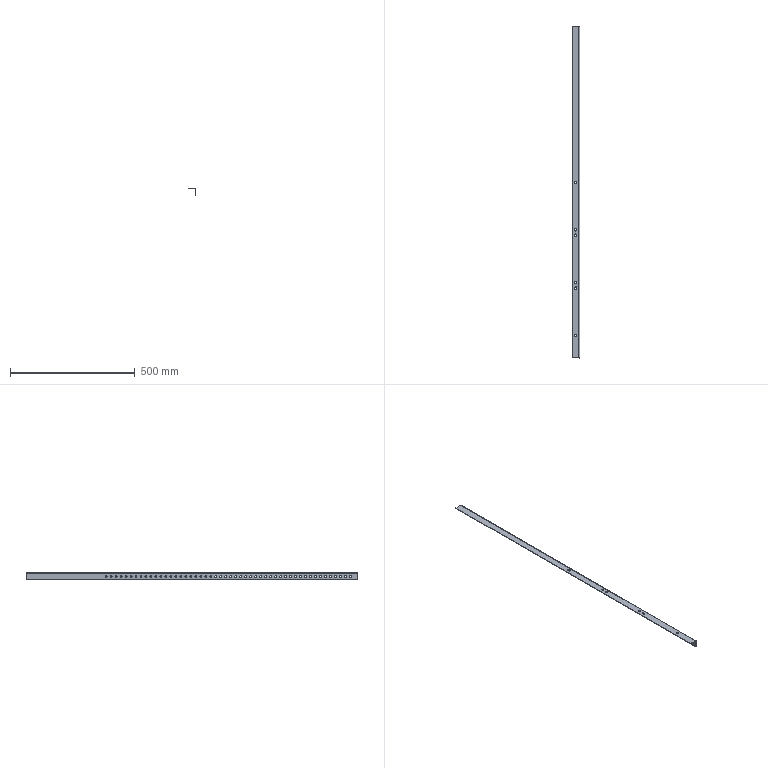Component | SolidWorks | BoxWelding-1_SupportPlate3.2-1 | 1 solid | 134 faces | box 31 x 1331 x 31 mm | volume 149430 mm3 | cylinder 114 | plane 20 | commonest cylinder face diameters 8 x100 6.4 x12 10 x1 6 x1
build123d program:
from build123d import *

# Parameters (mm, degrees)
EXTRUDE_THIN1_DEPTH = 665.5
SKETCH2_R           = 4
CUT_EXTRUDE1_DEPTH  = 10
CUT_EXTRUDE2_DEPTH  = 10


with BuildPart() as part:
    # Sketch1 → Extrude-Thin1 (new, symmetric)
    with BuildSketch(Plane.XY):
        with BuildLine():
            Line((-1, 30), (-1, 4))
            ThreePointArc((-1, 4), (-1.879, 1.879), (-4, 1))
            Line((-4, 1), (-30, 1))
            Line((-30, 1), (-30, -1))
            Line((-30, -1), (-4, -1))
            ThreePointArc((-4, -1), (-0.4645, 0.4645), (1, 4))
            Line((1, 4), (1, 30))
            Line((1, 30), (-1, 30))
        make_face()
    extrude(amount=EXTRUDE_THIN1_DEPTH, both=True)

    # Sketch2 → Cut-Extrude1 (cut)
    with BuildSketch(Plane.XZ.offset(1)):
        with Locations((-17, 635.5)):
            Circle(SKETCH2_R)
        with Locations((-17, 615.5)):
            Circle(SKETCH2_R)
        with Locations((-17, 595.5)):
            Circle(SKETCH2_R)
        with Locations((-17, 575.5)):
            Circle(SKETCH2_R)
        with Locations((-17, 555.5)):
            Circle(SKETCH2_R)
        with Locations((-17, 535.5)):
            Circle(SKETCH2_R)
        with Locations((-17, 515.5)):
            Circle(SKETCH2_R)
        with Locations((-17, 495.5)):
            Circle(SKETCH2_R)
        with Locations((-17, 475.5)):
            Circle(SKETCH2_R)
        with Locations((-17, 455.5)):
            Circle(SKETCH2_R)
        with Locations((-17, 435.5)):
            Circle(SKETCH2_R)
        with Locations((-17, 415.5)):
            Circle(SKETCH2_R)
        with Locations((-17, 395.5)):
            Circle(SKETCH2_R)
        with Locations((-17, 375.5)):
            Circle(SKETCH2_R)
        with Locations((-17, 355.5)):
            Circle(SKETCH2_R)
        with Locations((-17, 335.5)):
            Circle(SKETCH2_R)
        with Locations((-17, 315.5)):
            Circle(SKETCH2_R)
        with Locations((-17, 295.5)):
            Circle(SKETCH2_R)
        with Locations((-17, 275.5)):
            Circle(SKETCH2_R)
        with Locations((-17, 255.5)):
            Circle(SKETCH2_R)
        with Locations((-17, 235.5)):
            Circle(SKETCH2_R)
        with Locations((-17, 215.5)):
            Circle(SKETCH2_R)
        with Locations((-17, 195.5)):
            Circle(SKETCH2_R)
        with Locations((-17, 175.5)):
            Circle(SKETCH2_R)
        with Locations((-17, 155.5)):
            Circle(SKETCH2_R)
        with Locations((-17, 135.5)):
            Circle(SKETCH2_R)
        with Locations((-17, 115.5)):
            Circle(SKETCH2_R)
        with Locations((-17, 95.5)):
            Circle(SKETCH2_R)
        with Locations((-17, 75.5)):
            Circle(SKETCH2_R)
        with Locations((-17, 55.5)):
            Circle(SKETCH2_R)
        with Locations((-17, 35.5)):
            Circle(SKETCH2_R)
        with Locations((-17, 15.5)):
            Circle(SKETCH2_R)
        with Locations((-17, -4.5)):
            Circle(SKETCH2_R)
        with Locations((-17, -24.5)):
            Circle(SKETCH2_R)
        with Locations((-17, -44.5)):
            Circle(SKETCH2_R)
        with Locations((-17, -64.5)):
            Circle(SKETCH2_R)
        with Locations((-17, -84.5)):
            Circle(SKETCH2_R)
        with Locations((-17, -104.5)):
            Circle(SKETCH2_R)
        with Locations((-17, -124.5)):
            Circle(SKETCH2_R)
        with Locations((-17, -144.5)):
            Circle(SKETCH2_R)
        with Locations((-17, -164.5)):
            Circle(SKETCH2_R)
        with Locations((-17, -184.5)):
            Circle(SKETCH2_R)
        with Locations((-17, -204.5)):
            Circle(SKETCH2_R)
        with Locations((-17, -224.5)):
            Circle(SKETCH2_R)
        with Locations((-17, -244.5)):
            Circle(SKETCH2_R)
        with Locations((-17, -264.5)):
            Circle(SKETCH2_R)
        with Locations((-17, -284.5)):
            Circle(SKETCH2_R)
        with Locations((-17, -304.5)):
            Circle(SKETCH2_R)
        with Locations((-17, -324.5)):
            Circle(SKETCH2_R)
        with Locations((-17, -344.5)):
            Circle(SKETCH2_R)
    extrude(amount=-CUT_EXTRUDE1_DEPTH, mode=Mode.SUBTRACT)

    # Sketch3 → Cut-Extrude2 (cut)
    with BuildSketch(Plane(origin=(1, 0, 0), x_dir=(0, 0, -1), z_dir=(1, 0, 0))):
        with BuildLine():
            Line((-577.5, 19.2), (-573.5, 19.2))
            ThreePointArc((-573.5, 19.2), (-570.3, 16), (-573.5, 12.8))
            Line((-573.5, 12.8), (-577.5, 12.8))
            ThreePointArc((-577.5, 12.8), (-580.7, 16), (-577.5, 19.2))
        make_face()
        with BuildLine():
            Line((-387.5, 19.2), (-383.5, 19.2))
            ThreePointArc((-383.5, 19.2), (-380.3, 16), (-383.5, 12.8))
            Line((-383.5, 12.8), (-387.5, 12.8))
            ThreePointArc((-387.5, 12.8), (-390.7, 16), (-387.5, 19.2))
        make_face()
        with BuildLine():
            Line((-175.5, 19.2), (-171.5, 19.2))
            ThreePointArc((-171.5, 19.2), (-168.3, 16), (-171.5, 12.8))
            Line((-171.5, 12.8), (-175.5, 12.8))
            ThreePointArc((-175.5, 12.8), (-178.7, 16), (-175.5, 19.2))
        make_face()
        with BuildLine():
            Line((36.5, 19.2), (40.5, 19.2))
            ThreePointArc((40.5, 19.2), (43.7, 16), (40.5, 12.8))
            Line((40.5, 12.8), (36.5, 12.8))
            ThreePointArc((36.5, 12.8), (33.3, 16), (36.5, 19.2))
        make_face()
        with BuildLine():
            Line((-153.5, 19.2), (-149.5, 19.2))
            ThreePointArc((-149.5, 19.2), (-146.3, 16), (-149.5, 12.8))
            Line((-149.5, 12.8), (-153.5, 12.8))
            ThreePointArc((-153.5, 12.8), (-156.7, 16), (-153.5, 19.2))
        make_face()
        with BuildLine():
            Line((-365.5, 19.2), (-361.5, 19.2))
            ThreePointArc((-361.5, 19.2), (-358.3, 16), (-361.5, 12.8))
            Line((-361.5, 12.8), (-365.5, 12.8))
            ThreePointArc((-365.5, 12.8), (-368.7, 16), (-365.5, 19.2))
        make_face()
    extrude(amount=-CUT_EXTRUDE2_DEPTH, mode=Mode.SUBTRACT)


solid = part.part

# Placed as in the assembly
solid = solid.moved(Location((270.622, 621.001, 345.013), (90, 0, 90)))